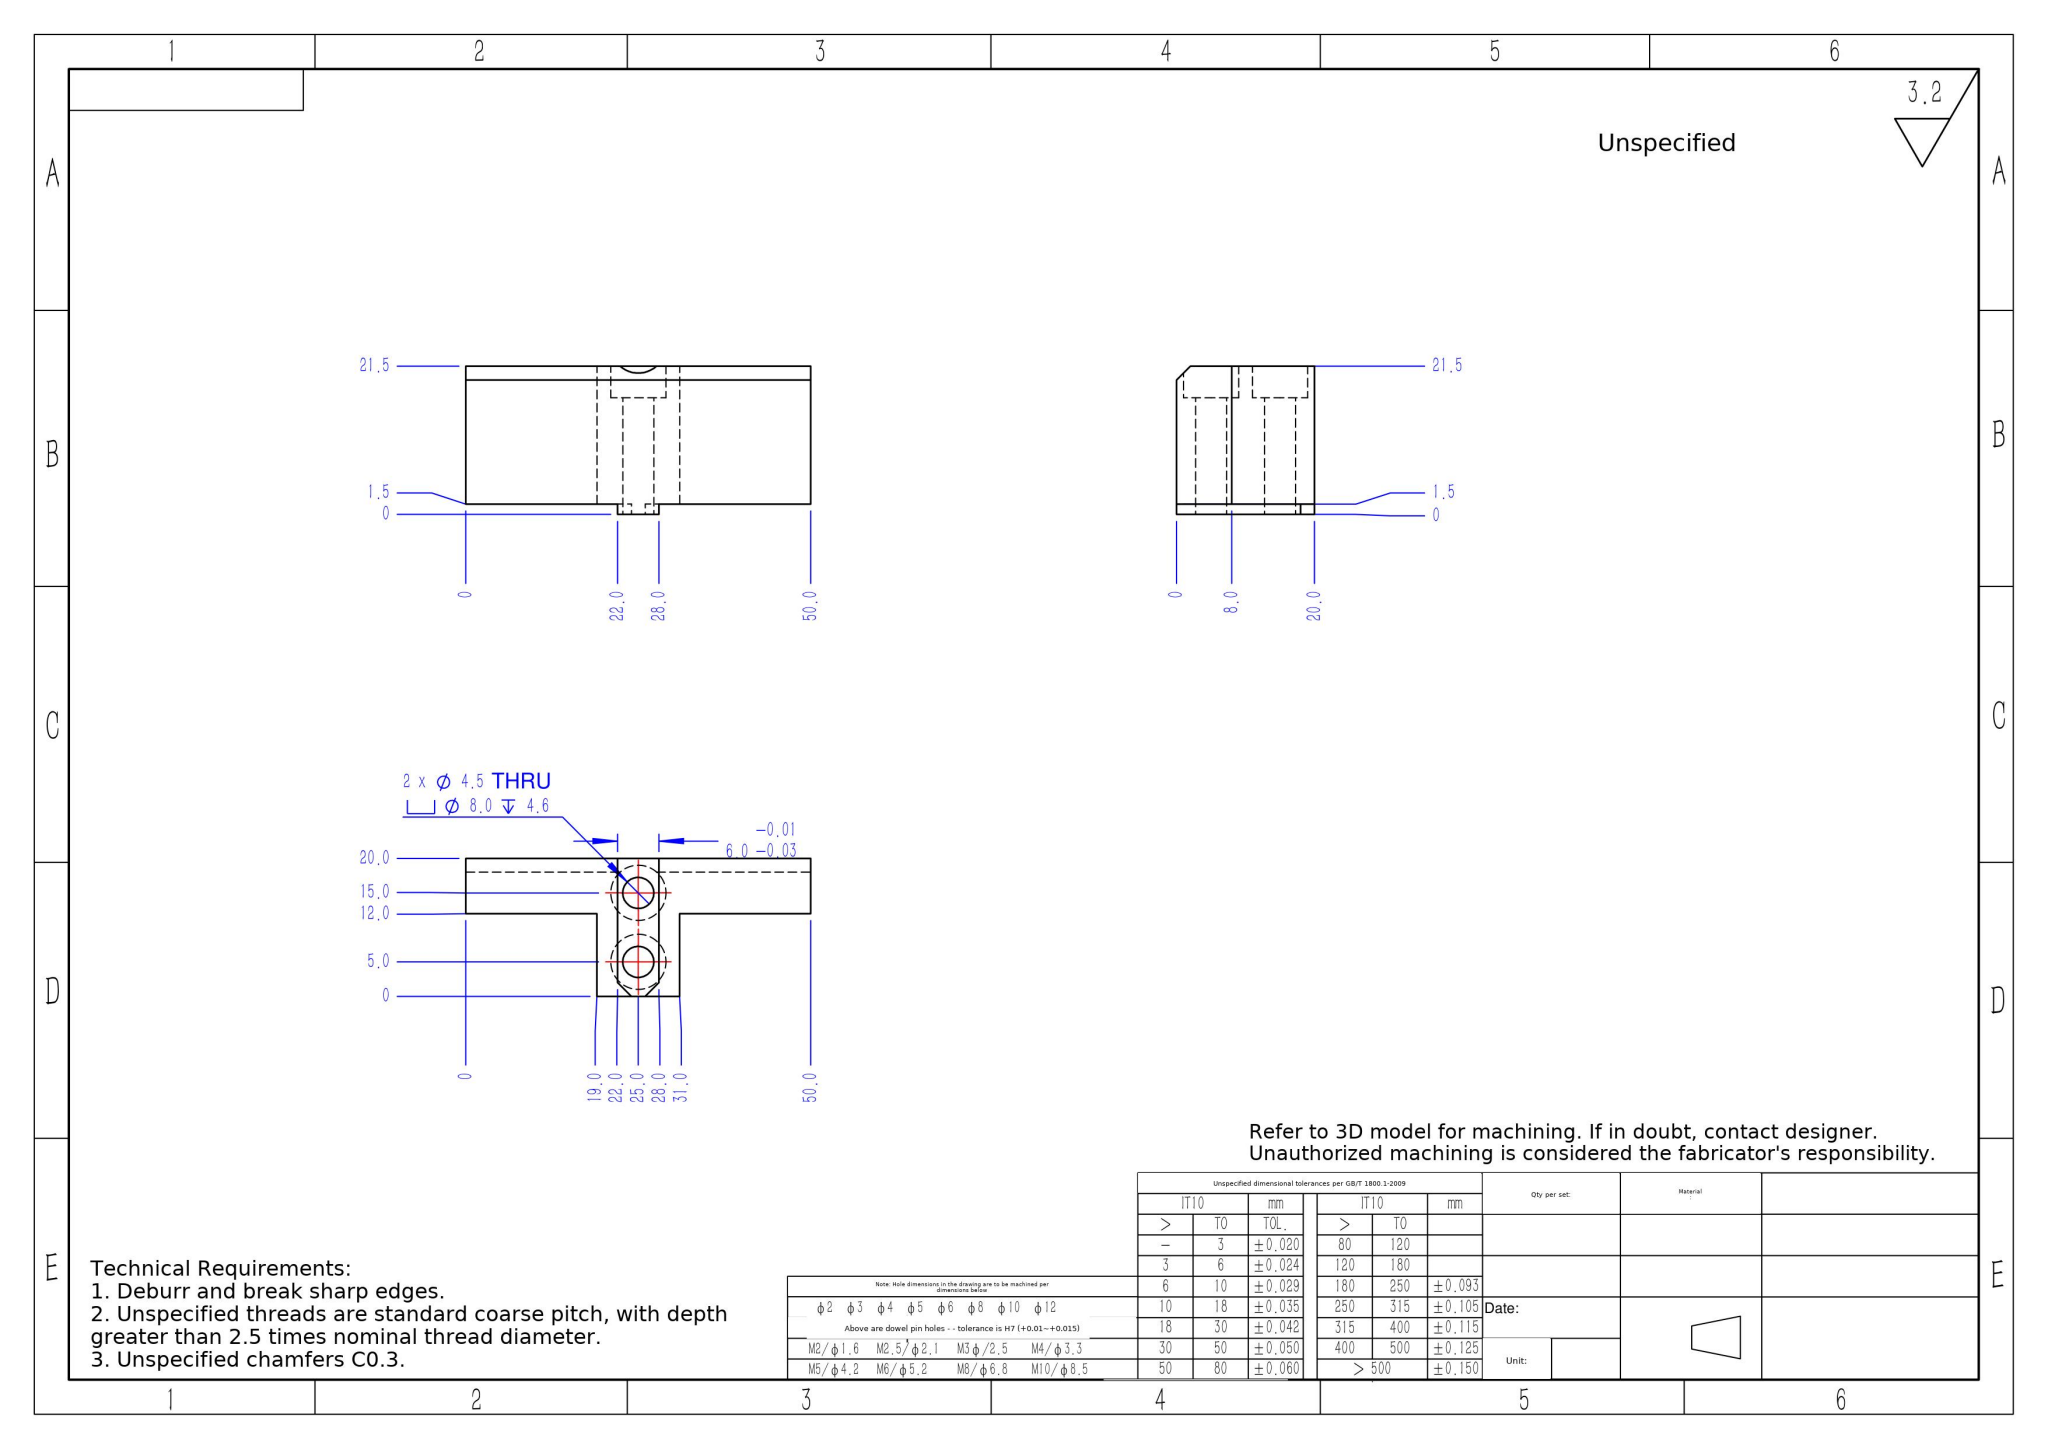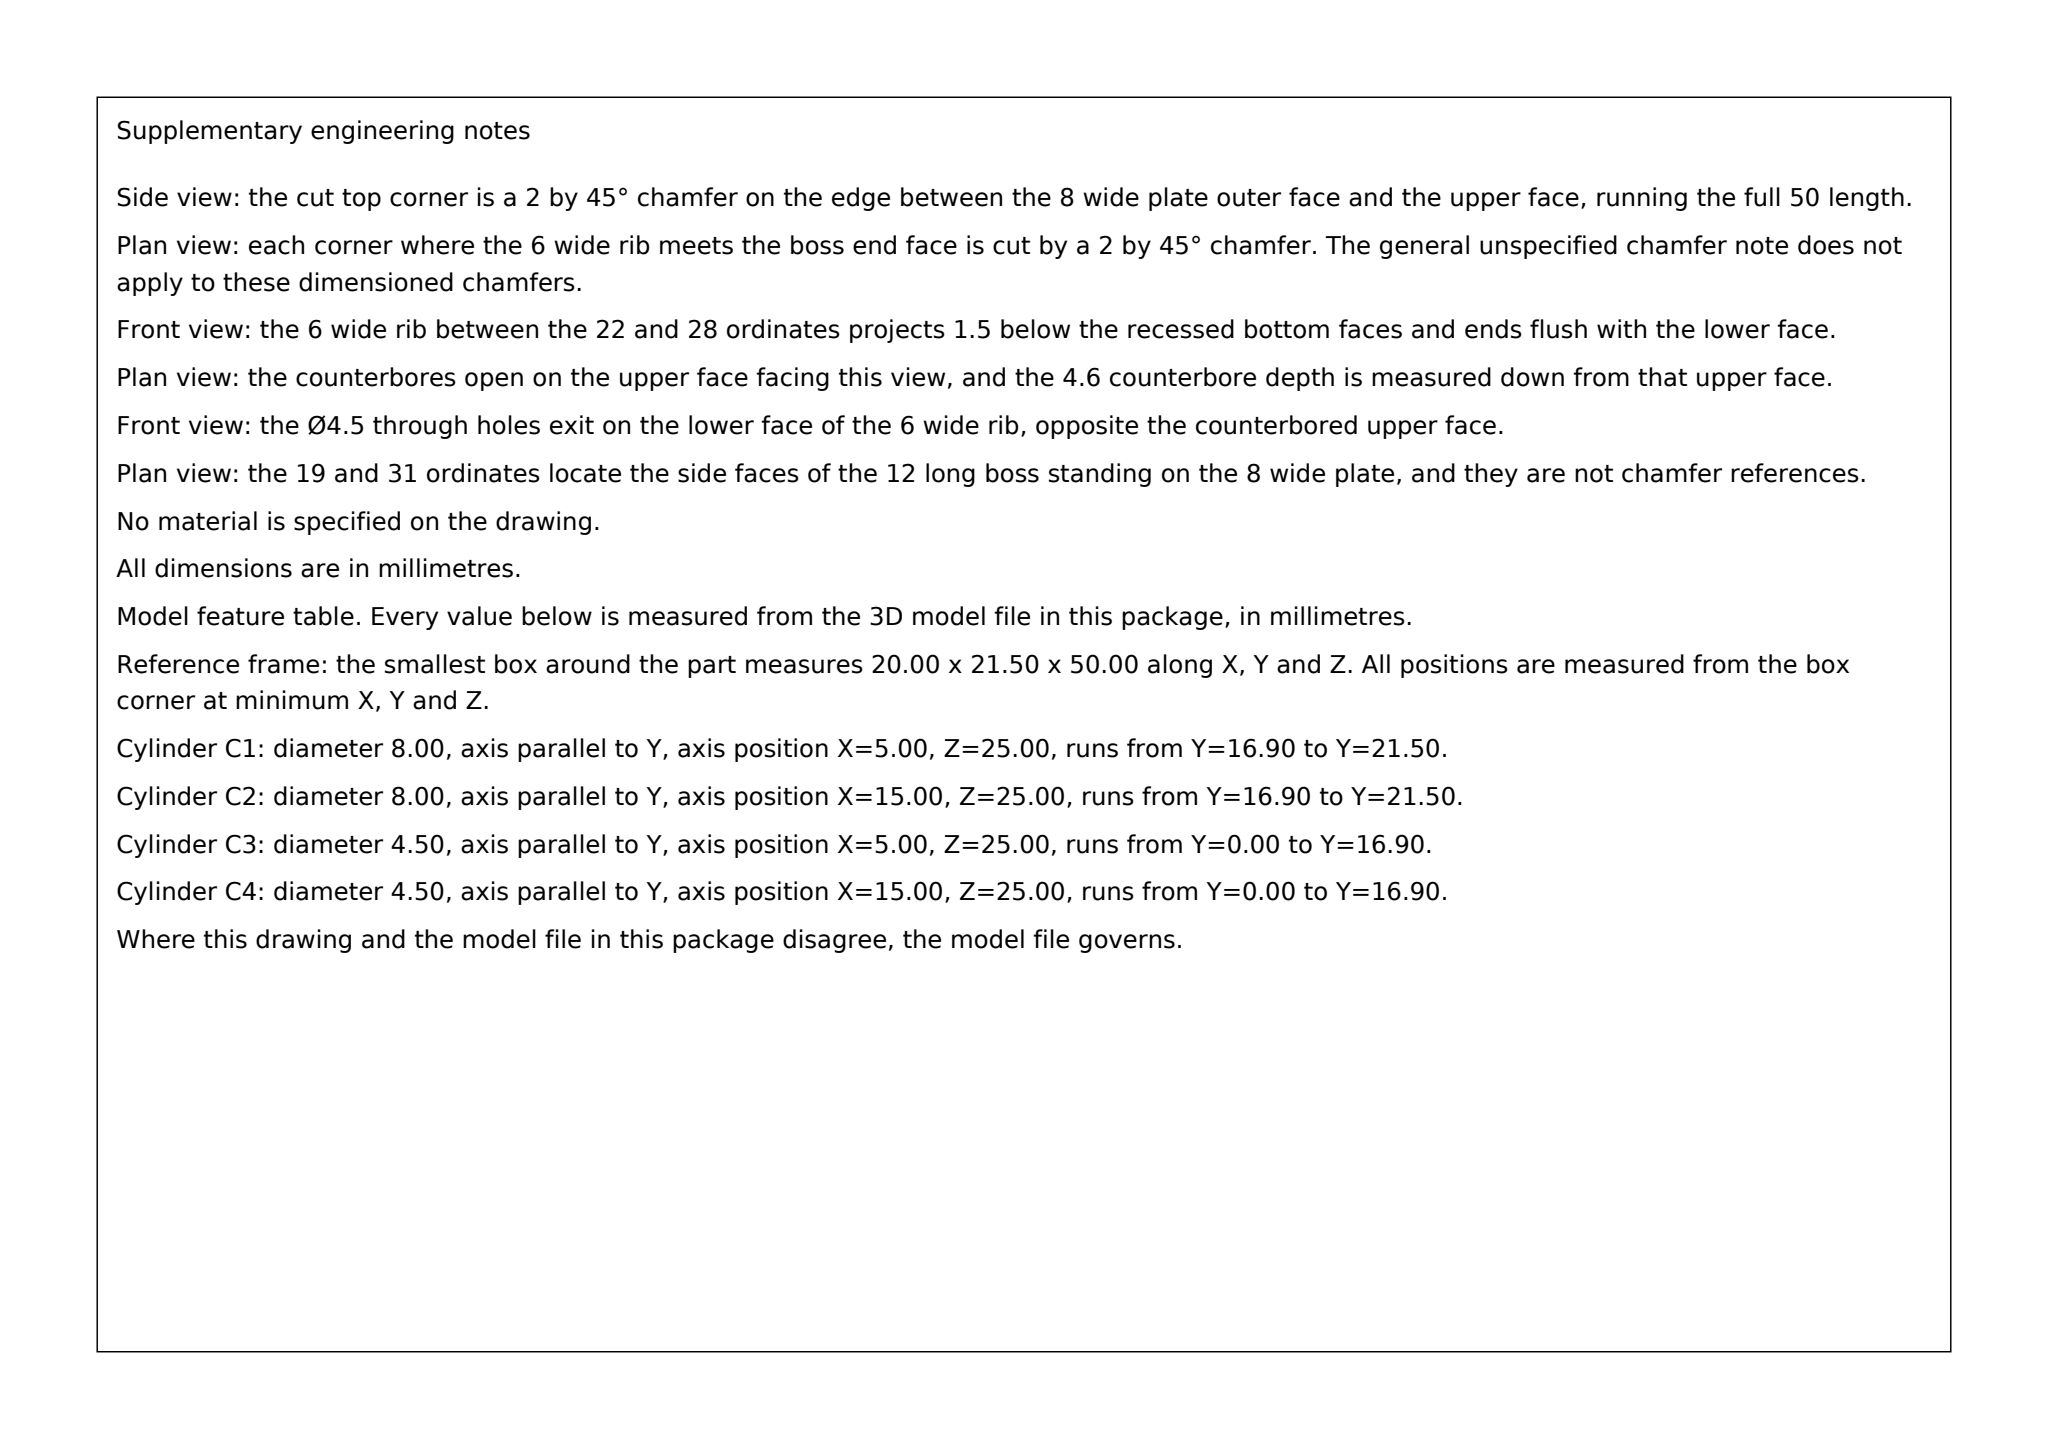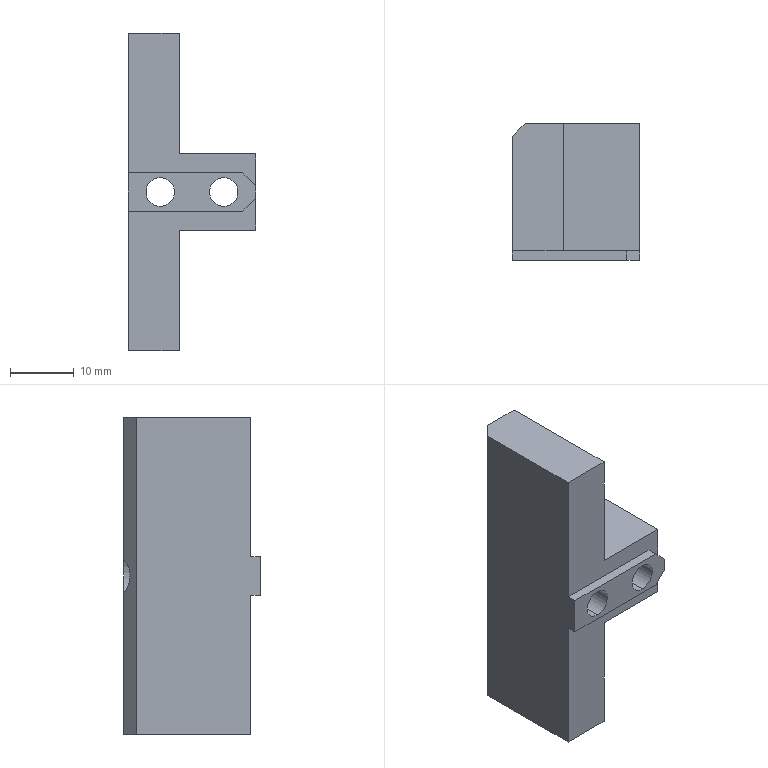Part | SolidWorks | mm | 1 solid | 27 faces | box 20 x 21.5 x 50 mm | volume 9955 mm3 | plane 19 | cylinder 8 | commonest cylinder face diameters 8 x4 4.5 x4
Drawing notes:
2X C2 ON 6 WIDE SLOT ENDS AT 18.0, Z 22.0 & 28.0 | from the solid: inclined_planes 45/90/45 at bbox_from [18,0,22] & [18,0,26], size 2x1.5x2 (two chamfers, 2mm leg = C2) on slot bounded by z=22.0/28.0 faces and x=18 end
STEP:
#1=CARTESIAN_POINT('',(15.,16.9,-29.));
#2=VERTEX_POINT('',#1);
#3=CARTESIAN_POINT('',(15.,16.9,-21.));
#4=VERTEX_POINT('',#3);
#5=CARTESIAN_POINT('',(15.,16.9,-25.));
#6=DIRECTION('',(0.,1.,0.));
#7=DIRECTION('',(0.,0.,1.));
#8=AXIS2_PLACEMENT_3D('',#5,#6,#7);
#9=CIRCLE('',#8,4.);
#10=EDGE_CURVE('',#2,#4,#9,.T.);
#11=ORIENTED_EDGE('',*,*,#10,.F.);
#12=CARTESIAN_POINT('',(15.,21.5,-29.));
#13=VERTEX_POINT('',#12);
#14=CARTESIAN_POINT('',(15.,21.5,-29.));
#15=DIRECTION('',(0.,1.,0.));
#16=VECTOR('',#15,1000.);
#17=LINE('',#14,#16);
#18=EDGE_CURVE('',#2,#13,#17,.T.);
#19=ORIENTED_EDGE('',*,*,#18,.T.);
#20=CARTESIAN_POINT('',(15.,21.5,-21.));
#21=VERTEX_POINT('',#20);
#22=CARTESIAN_POINT('',(15.,21.5,-25.));
#23=DIRECTION('',(0.,1.,0.));
#24=DIRECTION('',(0.,0.,1.));
#25=AXIS2_PLACEMENT_3D('',#22,#23,#24);
#26=CIRCLE('',#25,4.);
#27=EDGE_CURVE('',#13,#21,#26,.T.);
#28=ORIENTED_EDGE('',*,*,#27,.T.);
#29=CARTESIAN_POINT('',(15.,21.5,-21.));
#30=DIRECTION('',(0.,1.,0.));
#31=VECTOR('',#30,1000.);
#32=LINE('',#29,#31);
#33=EDGE_CURVE('',#4,#21,#32,.T.);
#34=ORIENTED_EDGE('',*,*,#33,.F.);
#35=EDGE_LOOP('',(#11,#19,#28,#34));
#36=FACE_OUTER_BOUND('',#35,.T.);
#37=CARTESIAN_POINT('',(15.,21.5,-25.));
#38=DIRECTION('',(0.,1.,0.));
#39=DIRECTION('',(0.,0.,1.));
#40=AXIS2_PLACEMENT_3D('',#37,#38,#39);
#41=CYLINDRICAL_SURFACE('',#40,4.);
#42=ADVANCED_FACE('',(#36),#41,.F.);
#43=CARTESIAN_POINT('',(15.,0.,-27.25));
#44=VERTEX_POINT('',#43);
#45=CARTESIAN_POINT('',(15.,0.,-22.75));
#46=VERTEX_POINT('',#45);
#47=CARTESIAN_POINT('',(15.,0.,-25.));
#48=DIRECTION('',(0.,1.,0.));
#49=DIRECTION('',(0.,0.,1.));
#50=AXIS2_PLACEMENT_3D('',#47,#48,#49);
#51=CIRCLE('',#50,2.25);
#52=EDGE_CURVE('',#44,#46,#51,.T.);
#53=ORIENTED_EDGE('',*,*,#52,.F.);
#54=CARTESIAN_POINT('',(15.,16.9,-27.25));
#55=VERTEX_POINT('',#54);
#56=CARTESIAN_POINT('',(15.,21.5,-27.25));
#57=DIRECTION('',(0.,1.,0.));
#58=VECTOR('',#57,1000.);
#59=LINE('',#56,#58);
#60=EDGE_CURVE('',#44,#55,#59,.T.);
#61=ORIENTED_EDGE('',*,*,#60,.T.);
#62=CARTESIAN_POINT('',(15.,16.9,-22.75));
#63=VERTEX_POINT('',#62);
#64=CARTESIAN_POINT('',(15.,16.9,-25.));
#65=DIRECTION('',(0.,1.,0.));
#66=DIRECTION('',(0.,0.,1.));
#67=AXIS2_PLACEMENT_3D('',#64,#65,#66);
#68=CIRCLE('',#67,2.25);
#69=EDGE_CURVE('',#55,#63,#68,.T.);
#70=ORIENTED_EDGE('',*,*,#69,.T.);
#71=CARTESIAN_POINT('',(15.,21.5,-22.75));
#72=DIRECTION('',(0.,1.,0.));
#73=VECTOR('',#72,1000.);
#74=LINE('',#71,#73);
#75=EDGE_CURVE('',#46,#63,#74,.T.);
#76=ORIENTED_EDGE('',*,*,#75,.F.);
#77=EDGE_LOOP('',(#53,#61,#70,#76));
#78=FACE_OUTER_BOUND('',#77,.T.);
#79=CARTESIAN_POINT('',(15.,21.5,-25.));
#80=DIRECTION('',(0.,1.,0.));
#81=DIRECTION('',(0.,0.,1.));
#82=AXIS2_PLACEMENT_3D('',#79,#80,#81);
#83=CYLINDRICAL_SURFACE('',#82,2.25);
#84=ADVANCED_FACE('',(#78),#83,.F.);
#85=CARTESIAN_POINT('',(5.,16.9,-29.));
#86=VERTEX_POINT('',#85);
#87=CARTESIAN_POINT('',(5.,16.9,-21.));
#88=VERTEX_POINT('',#87);
#89=CARTESIAN_POINT('',(5.,16.9,-25.));
#90=DIRECTION('',(0.,1.,0.));
#91=DIRECTION('',(0.,0.,1.));
#92=AXIS2_PLACEMENT_3D('',#89,#90,#91);
#93=CIRCLE('',#92,4.);
#94=EDGE_CURVE('',#86,#88,#93,.T.);
#95=ORIENTED_EDGE('',*,*,#94,.F.);
#96=CARTESIAN_POINT('',(5.,21.5,-29.));
#97=VERTEX_POINT('',#96);
#98=CARTESIAN_POINT('',(5.,21.5,-29.));
#99=DIRECTION('',(0.,1.,0.));
#100=VECTOR('',#99,1000.);
#101=LINE('',#98,#100);
#102=EDGE_CURVE('',#86,#97,#101,.T.);
#103=ORIENTED_EDGE('',*,*,#102,.T.);
#104=CARTESIAN_POINT('',(2.,21.5,-27.646));
#105=VERTEX_POINT('',#104);
#106=CARTESIAN_POINT('',(5.,21.5,-25.));
#107=DIRECTION('',(0.,1.,0.));
#108=DIRECTION('',(0.,0.,1.));
#109=AXIS2_PLACEMENT_3D('',#106,#107,#108);
#110=CIRCLE('',#109,4.);
#111=EDGE_CURVE('',#97,#105,#110,.T.);
#112=ORIENTED_EDGE('',*,*,#111,.T.);
#113=CARTESIAN_POINT('',(2.,21.5,-22.354));
#114=VERTEX_POINT('',#113);
#115=CARTESIAN_POINT('',(2.,21.5,-27.646));
#116=CARTESIAN_POINT('',(0.6,20.1,-26.058));
#117=CARTESIAN_POINT('',(0.6,20.1,-23.942));
#118=CARTESIAN_POINT('',(2.,21.5,-22.354));
#119=(BOUNDED_CURVE()B_SPLINE_CURVE(3,(#115,#116,#117,#118),.UNSPECIFIED.,.F.,.F.)B_SPLINE_CURVE_WITH_KNOTS((4,4),(2.419,3.864),.UNSPECIFIED.)CURVE()GEOMETRIC_REPRESENTATION_ITEM()RATIONAL_B_SPLINE_CURVE((1.,0.8333,0.8333,1.))REPRESENTATION_ITEM(''));
#120=EDGE_CURVE('',#105,#114,#119,.T.);
#121=ORIENTED_EDGE('',*,*,#120,.T.);
#122=CARTESIAN_POINT('',(5.,21.5,-21.));
#123=VERTEX_POINT('',#122);
#124=CARTESIAN_POINT('',(5.,21.5,-25.));
#125=DIRECTION('',(0.,1.,0.));
#126=DIRECTION('',(0.,0.,1.));
#127=AXIS2_PLACEMENT_3D('',#124,#125,#126);
#128=CIRCLE('',#127,4.);
#129=EDGE_CURVE('',#114,#123,#128,.T.);
#130=ORIENTED_EDGE('',*,*,#129,.T.);
#131=CARTESIAN_POINT('',(5.,21.5,-21.));
#132=DIRECTION('',(0.,1.,0.));
#133=VECTOR('',#132,1000.);
#134=LINE('',#131,#133);
#135=EDGE_CURVE('',#88,#123,#134,.T.);
#136=ORIENTED_EDGE('',*,*,#135,.F.);
#137=EDGE_LOOP('',(#95,#103,#112,#121,#130,#136));
#138=FACE_OUTER_BOUND('',#137,.T.);
#139=CARTESIAN_POINT('',(5.,21.5,-25.));
#140=DIRECTION('',(0.,1.,0.));
#141=DIRECTION('',(0.,0.,1.));
#142=AXIS2_PLACEMENT_3D('',#139,#140,#141);
#143=CYLINDRICAL_SURFACE('',#142,4.);
#144=ADVANCED_FACE('',(#138),#143,.F.);
#145=CARTESIAN_POINT('',(5.,0.,-27.25));
#146=VERTEX_POINT('',#145);
#147=CARTESIAN_POINT('',(5.,0.,-22.75));
#148=VERTEX_POINT('',#147);
#149=CARTESIAN_POINT('',(5.,0.,-25.));
#150=DIRECTION('',(0.,1.,0.));
#151=DIRECTION('',(0.,0.,1.));
#152=AXIS2_PLACEMENT_3D('',#149,#150,#151);
#153=CIRCLE('',#152,2.25);
#154=EDGE_CURVE('',#146,#148,#153,.T.);
#155=ORIENTED_EDGE('',*,*,#154,.F.);
#156=CARTESIAN_POINT('',(5.,16.9,-27.25));
#157=VERTEX_POINT('',#156);
#158=CARTESIAN_POINT('',(5.,21.5,-27.25));
#159=DIRECTION('',(0.,1.,0.));
#160=VECTOR('',#159,1000.);
#161=LINE('',#158,#160);
#162=EDGE_CURVE('',#146,#157,#161,.T.);
#163=ORIENTED_EDGE('',*,*,#162,.T.);
#164=CARTESIAN_POINT('',(5.,16.9,-22.75));
#165=VERTEX_POINT('',#164);
#166=CARTESIAN_POINT('',(5.,16.9,-25.));
#167=DIRECTION('',(0.,1.,0.));
#168=DIRECTION('',(0.,0.,1.));
#169=AXIS2_PLACEMENT_3D('',#166,#167,#168);
#170=CIRCLE('',#169,2.25);
#171=EDGE_CURVE('',#157,#165,#170,.T.);
#172=ORIENTED_EDGE('',*,*,#171,.T.);
#173=CARTESIAN_POINT('',(5.,21.5,-22.75));
#174=DIRECTION('',(0.,1.,0.));
#175=VECTOR('',#174,1000.);
#176=LINE('',#173,#175);
#177=EDGE_CURVE('',#148,#165,#176,.T.);
#178=ORIENTED_EDGE('',*,*,#177,.F.);
#179=EDGE_LOOP('',(#155,#163,#172,#178));
#180=FACE_OUTER_BOUND('',#179,.T.);
#181=CARTESIAN_POINT('',(5.,21.5,-25.));
#182=DIRECTION('',(0.,1.,0.));
#183=DIRECTION('',(0.,0.,1.));
#184=AXIS2_PLACEMENT_3D('',#181,#182,#183);
#185=CYLINDRICAL_SURFACE('',#184,2.25);
#186=ADVANCED_FACE('',(#180),#185,.F.);
#187=CARTESIAN_POINT('',(0.,19.5,0.));
#188=VERTEX_POINT('',#187);
#189=CARTESIAN_POINT('',(0.,1.5,0.));
#190=VERTEX_POINT('',#189);
#191=CARTESIAN_POINT('',(0.,21.5,0.));
#192=DIRECTION('',(0.,-1.,0.));
#193=VECTOR('',#192,1000.);
#194=LINE('',#191,#193);
#195=EDGE_CURVE('',#188,#190,#194,.T.);
#196=ORIENTED_EDGE('',*,*,#195,.F.);
#197=CARTESIAN_POINT('',(0.,19.5,-50.));
#198=VERTEX_POINT('',#197);
#199=CARTESIAN_POINT('',(0.,19.5,0.));
#200=DIRECTION('',(0.,0.,-1.));
#201=VECTOR('',#200,1000.);
#202=LINE('',#199,#201);
#203=EDGE_CURVE('',#188,#198,#202,.T.);
#204=ORIENTED_EDGE('',*,*,#203,.T.);
#205=CARTESIAN_POINT('',(0.,1.5,-50.));
#206=VERTEX_POINT('',#205);
#207=CARTESIAN_POINT('',(0.,21.5,-50.));
#208=DIRECTION('',(0.,-1.,0.));
#209=VECTOR('',#208,1000.);
#210=LINE('',#207,#209);
#211=EDGE_CURVE('',#198,#206,#210,.T.);
#212=ORIENTED_EDGE('',*,*,#211,.T.);
#213=CARTESIAN_POINT('',(0.,1.5,-28.));
#214=VERTEX_POINT('',#213);
#215=CARTESIAN_POINT('',(0.,1.5,-28.));
#216=DIRECTION('',(0.,0.,1.));
#217=VECTOR('',#216,1000.);
#218=LINE('',#215,#217);
#219=EDGE_CURVE('',#206,#214,#218,.T.);
#220=ORIENTED_EDGE('',*,*,#219,.T.);
#221=CARTESIAN_POINT('',(0.,0.,-28.));
#222=VERTEX_POINT('',#221);
#223=CARTESIAN_POINT('',(0.,1.5,-28.));
#224=DIRECTION('',(0.,-1.,0.));
#225=VECTOR('',#224,1000.);
#226=LINE('',#223,#225);
#227=EDGE_CURVE('',#214,#222,#226,.T.);
#228=ORIENTED_EDGE('',*,*,#227,.T.);
#229=CARTESIAN_POINT('',(0.,0.,-22.));
#230=VERTEX_POINT('',#229);
#231=CARTESIAN_POINT('',(0.,0.,0.));
#232=DIRECTION('',(0.,0.,1.));
#233=VECTOR('',#232,1000.);
#234=LINE('',#231,#233);
#235=EDGE_CURVE('',#222,#230,#234,.T.);
#236=ORIENTED_EDGE('',*,*,#235,.T.);
#237=CARTESIAN_POINT('',(0.,1.5,-22.));
#238=VERTEX_POINT('',#237);
#239=CARTESIAN_POINT('',(0.,1.5,-22.));
#240=DIRECTION('',(0.,1.,0.));
#241=VECTOR('',#240,1000.);
#242=LINE('',#239,#241);
#243=EDGE_CURVE('',#230,#238,#242,.T.);
#244=ORIENTED_EDGE('',*,*,#243,.T.);
#245=CARTESIAN_POINT('',(0.,1.5,2.879));
#246=DIRECTION('',(0.,0.,1.));
#247=VECTOR('',#246,1000.);
#248=LINE('',#245,#247);
#249=EDGE_CURVE('',#238,#190,#248,.T.);
#250=ORIENTED_EDGE('',*,*,#249,.T.);
#251=EDGE_LOOP('',(#196,#204,#212,#220,#228,#236,#244,#250));
#252=FACE_OUTER_BOUND('',#251,.T.);
#253=CARTESIAN_POINT('',(0.,21.5,0.));
#254=DIRECTION('',(1.,0.,0.));
#255=DIRECTION('',(0.,0.,-1.));
#256=AXIS2_PLACEMENT_3D('',#253,#254,#255);
#257=PLANE('',#256);
#258=ADVANCED_FACE('',(#252),#257,.F.);
#259=CARTESIAN_POINT('',(2.,21.5,0.));
#260=VERTEX_POINT('',#259);
#261=CARTESIAN_POINT('',(8.,21.5,0.));
#262=VERTEX_POINT('',#261);
#263=CARTESIAN_POINT('',(0.,21.5,0.));
#264=DIRECTION('',(1.,0.,0.));
#265=VECTOR('',#264,1000.);
#266=LINE('',#263,#265);
#267=EDGE_CURVE('',#260,#262,#266,.T.);
#268=ORIENTED_EDGE('',*,*,#267,.F.);
#269=CARTESIAN_POINT('',(2.,21.5,0.));
#270=DIRECTION('',(-0.7071,-0.7071,0.));
#271=VECTOR('',#270,1000.);
#272=LINE('',#269,#271);
#273=EDGE_CURVE('',#260,#188,#272,.T.);
#274=ORIENTED_EDGE('',*,*,#273,.T.);
#275=ORIENTED_EDGE('',*,*,#195,.T.);
#276=CARTESIAN_POINT('',(8.,1.5,0.));
#277=VERTEX_POINT('',#276);
#278=CARTESIAN_POINT('',(0.,1.5,0.));
#279=DIRECTION('',(1.,0.,0.));
#280=VECTOR('',#279,1000.);
#281=LINE('',#278,#280);
#282=EDGE_CURVE('',#190,#277,#281,.T.);
#283=ORIENTED_EDGE('',*,*,#282,.T.);
#284=CARTESIAN_POINT('',(8.,21.5,0.));
#285=DIRECTION('',(0.,1.,0.));
#286=VECTOR('',#285,1000.);
#287=LINE('',#284,#286);
#288=EDGE_CURVE('',#277,#262,#287,.T.);
#289=ORIENTED_EDGE('',*,*,#288,.T.);
#290=EDGE_LOOP('',(#268,#274,#275,#283,#289));
#291=FACE_OUTER_BOUND('',#290,.T.);
#292=CARTESIAN_POINT('',(0.,21.5,0.));
#293=DIRECTION('',(0.,0.,-1.));
#294=DIRECTION('',(-1.,0.,0.));
#295=AXIS2_PLACEMENT_3D('',#292,#293,#294);
#296=PLANE('',#295);
#297=ADVANCED_FACE('',(#291),#296,.F.);
#298=CARTESIAN_POINT('',(20.,1.5,-24.));
#299=VERTEX_POINT('',#298);
#300=CARTESIAN_POINT('',(20.,1.5,-19.));
#301=VERTEX_POINT('',#300);
#302=CARTESIAN_POINT('',(20.,1.5,2.879));
#303=DIRECTION('',(0.,0.,1.));
#304=VECTOR('',#303,1000.);
#305=LINE('',#302,#304);
#306=EDGE_CURVE('',#299,#301,#305,.T.);
#307=ORIENTED_EDGE('',*,*,#306,.F.);
#308=CARTESIAN_POINT('',(20.,0.,-24.));
#309=VERTEX_POINT('',#308);
#310=CARTESIAN_POINT('',(20.,21.5,-24.));
#311=DIRECTION('',(0.,-1.,0.));
#312=VECTOR('',#311,1000.);
#313=LINE('',#310,#312);
#314=EDGE_CURVE('',#299,#309,#313,.T.);
#315=ORIENTED_EDGE('',*,*,#314,.T.);
#316=CARTESIAN_POINT('',(20.,0.,-26.));
#317=VERTEX_POINT('',#316);
#318=CARTESIAN_POINT('',(20.,0.,0.));
#319=DIRECTION('',(0.,0.,-1.));
#320=VECTOR('',#319,1000.);
#321=LINE('',#318,#320);
#322=EDGE_CURVE('',#309,#317,#321,.T.);
#323=ORIENTED_EDGE('',*,*,#322,.T.);
#324=CARTESIAN_POINT('',(20.,1.5,-26.));
#325=VERTEX_POINT('',#324);
#326=CARTESIAN_POINT('',(20.,21.5,-26.));
#327=DIRECTION('',(0.,1.,-0.));
#328=VECTOR('',#327,1000.);
#329=LINE('',#326,#328);
#330=EDGE_CURVE('',#317,#325,#329,.T.);
#331=ORIENTED_EDGE('',*,*,#330,.T.);
#332=CARTESIAN_POINT('',(20.,1.5,-31.));
#333=VERTEX_POINT('',#332);
#334=CARTESIAN_POINT('',(20.,1.5,-28.));
#335=DIRECTION('',(0.,0.,1.));
#336=VECTOR('',#335,1000.);
#337=LINE('',#334,#336);
#338=EDGE_CURVE('',#333,#325,#337,.T.);
#339=ORIENTED_EDGE('',*,*,#338,.F.);
#340=CARTESIAN_POINT('',(20.,21.5,-31.));
#341=VERTEX_POINT('',#340);
#342=CARTESIAN_POINT('',(20.,21.5,-31.));
#343=DIRECTION('',(0.,1.,0.));
#344=VECTOR('',#343,1000.);
#345=LINE('',#342,#344);
#346=EDGE_CURVE('',#333,#341,#345,.T.);
#347=ORIENTED_EDGE('',*,*,#346,.T.);
#348=CARTESIAN_POINT('',(20.,21.5,-19.));
#349=VERTEX_POINT('',#348);
#350=CARTESIAN_POINT('',(20.,21.5,0.));
#351=DIRECTION('',(0.,0.,-1.));
#352=VECTOR('',#351,1000.);
#353=LINE('',#350,#352);
#354=EDGE_CURVE('',#349,#341,#353,.T.);
#355=ORIENTED_EDGE('',*,*,#354,.F.);
#356=CARTESIAN_POINT('',(20.,21.5,-19.));
#357=DIRECTION('',(0.,-1.,0.));
#358=VECTOR('',#357,1000.);
#359=LINE('',#356,#358);
#360=EDGE_CURVE('',#349,#301,#359,.T.);
#361=ORIENTED_EDGE('',*,*,#360,.T.);
#362=EDGE_LOOP('',(#307,#315,#323,#331,#339,#347,#355,#361));
#363=FACE_OUTER_BOUND('',#362,.T.);
#364=CARTESIAN_POINT('',(20.,21.5,0.));
#365=DIRECTION('',(-1.,0.,0.));
#366=DIRECTION('',(0.,0.,1.));
#367=AXIS2_PLACEMENT_3D('',#364,#365,#366);
#368=PLANE('',#367);
#369=ADVANCED_FACE('',(#363),#368,.F.);
#370=ORIENTED_EDGE('',*,*,#211,.F.);
#371=CARTESIAN_POINT('',(2.,21.5,-50.));
#372=VERTEX_POINT('',#371);
#373=CARTESIAN_POINT('',(2.,21.5,-50.));
#374=DIRECTION('',(0.7071,0.7071,0.));
#375=VECTOR('',#374,1000.);
#376=LINE('',#373,#375);
#377=EDGE_CURVE('',#198,#372,#376,.T.);
#378=ORIENTED_EDGE('',*,*,#377,.T.);
#379=CARTESIAN_POINT('',(8.,21.5,-50.));
#380=VERTEX_POINT('',#379);
#381=CARTESIAN_POINT('',(0.,21.5,-50.));
#382=DIRECTION('',(-1.,0.,0.));
#383=VECTOR('',#382,1000.);
#384=LINE('',#381,#383);
#385=EDGE_CURVE('',#380,#372,#384,.T.);
#386=ORIENTED_EDGE('',*,*,#385,.F.);
#387=CARTESIAN_POINT('',(8.,1.5,-50.));
#388=VERTEX_POINT('',#387);
#389=CARTESIAN_POINT('',(8.,21.5,-50.));
#390=DIRECTION('',(0.,-1.,0.));
#391=VECTOR('',#390,1000.);
#392=LINE('',#389,#391);
#393=EDGE_CURVE('',#380,#388,#392,.T.);
#394=ORIENTED_EDGE('',*,*,#393,.T.);
#395=CARTESIAN_POINT('',(0.,1.5,-50.));
#396=DIRECTION('',(-1.,0.,0.));
#397=VECTOR('',#396,1000.);
#398=LINE('',#395,#397);
#399=EDGE_CURVE('',#388,#206,#398,.T.);
#400=ORIENTED_EDGE('',*,*,#399,.T.);
#401=EDGE_LOOP('',(#370,#378,#386,#394,#400));
#402=FACE_OUTER_BOUND('',#401,.T.);
#403=CARTESIAN_POINT('',(0.,21.5,-50.));
#404=DIRECTION('',(0.,0.,1.));
#405=DIRECTION('',(1.,0.,0.));
#406=AXIS2_PLACEMENT_3D('',#403,#404,#405);
#407=PLANE('',#406);
#408=ADVANCED_FACE('',(#402),#407,.F.);
#409=CARTESIAN_POINT('',(15.,21.5,-25.));
#410=DIRECTION('',(0.,1.,0.));
#411=DIRECTION('',(0.,0.,1.));
#412=AXIS2_PLACEMENT_3D('',#409,#410,#411);
#413=CIRCLE('',#412,4.);
#414=EDGE_CURVE('',#21,#13,#413,.T.);
#415=ORIENTED_EDGE('',*,*,#414,.F.);
#416=ORIENTED_EDGE('',*,*,#27,.F.);
#417=EDGE_LOOP('',(#415,#416));
#418=FACE_BOUND('',#417,.T.);
#419=ORIENTED_EDGE('',*,*,#385,.T.);
#420=CARTESIAN_POINT('',(2.,21.5,0.));
#421=DIRECTION('',(0.,0.,1.));
#422=VECTOR('',#421,1000.);
#423=LINE('',#420,#422);
#424=EDGE_CURVE('',#372,#105,#423,.T.);
#425=ORIENTED_EDGE('',*,*,#424,.T.);
#426=ORIENTED_EDGE('',*,*,#111,.F.);
#427=CARTESIAN_POINT('',(5.,21.5,-25.));
#428=DIRECTION('',(0.,1.,0.));
#429=DIRECTION('',(0.,0.,1.));
#430=AXIS2_PLACEMENT_3D('',#427,#428,#429);
#431=CIRCLE('',#430,4.);
#432=EDGE_CURVE('',#123,#97,#431,.T.);
#433=ORIENTED_EDGE('',*,*,#432,.F.);
#434=ORIENTED_EDGE('',*,*,#129,.F.);
#435=CARTESIAN_POINT('',(2.,21.5,0.));
#436=DIRECTION('',(0.,0.,1.));
#437=VECTOR('',#436,1000.);
#438=LINE('',#435,#437);
#439=EDGE_CURVE('',#114,#260,#438,.T.);
#440=ORIENTED_EDGE('',*,*,#439,.T.);
#441=ORIENTED_EDGE('',*,*,#267,.T.);
#442=CARTESIAN_POINT('',(8.,21.5,-19.));
#443=VERTEX_POINT('',#442);
#444=CARTESIAN_POINT('',(8.,21.5,10.159));
#445=DIRECTION('',(0.,0.,1.));
#446=VECTOR('',#445,1000.);
#447=LINE('',#444,#446);
#448=EDGE_CURVE('',#443,#262,#447,.T.);
#449=ORIENTED_EDGE('',*,*,#448,.F.);
#450=CARTESIAN_POINT('',(8.,21.5,-19.));
#451=DIRECTION('',(-1.,0.,0.));
#452=VECTOR('',#451,1000.);
#453=LINE('',#450,#452);
#454=EDGE_CURVE('',#349,#443,#453,.T.);
#455=ORIENTED_EDGE('',*,*,#454,.F.);
#456=ORIENTED_EDGE('',*,*,#354,.T.);
#457=CARTESIAN_POINT('',(8.,21.5,-31.));
#458=VERTEX_POINT('',#457);
#459=CARTESIAN_POINT('',(8.,21.5,-31.));
#460=DIRECTION('',(1.,0.,0.));
#461=VECTOR('',#460,1000.);
#462=LINE('',#459,#461);
#463=EDGE_CURVE('',#458,#341,#462,.T.);
#464=ORIENTED_EDGE('',*,*,#463,.F.);
#465=CARTESIAN_POINT('',(8.,21.5,-50.245));
#466=DIRECTION('',(0.,0.,1.));
#467=VECTOR('',#466,1000.);
#468=LINE('',#465,#467);
#469=EDGE_CURVE('',#380,#458,#468,.T.);
#470=ORIENTED_EDGE('',*,*,#469,.F.);
#471=EDGE_LOOP('',(#419,#425,#426,#433,#434,#440,#441,#449,#455,#456,#464,#470));
#472=FACE_OUTER_BOUND('',#471,.T.);
#473=CARTESIAN_POINT('',(0.,21.5,0.));
#474=DIRECTION('',(0.,-1.,0.));
#475=DIRECTION('',(0.,0.,-1.));
#476=AXIS2_PLACEMENT_3D('',#473,#474,#475);
#477=PLANE('',#476);
#478=ADVANCED_FACE('',(#418,#472),#477,.F.);
#479=CARTESIAN_POINT('',(15.,0.,-25.));
#480=DIRECTION('',(0.,1.,0.));
#481=DIRECTION('',(0.,0.,1.));
#482=AXIS2_PLACEMENT_3D('',#479,#480,#481);
#483=CIRCLE('',#482,2.25);
#484=EDGE_CURVE('',#46,#44,#483,.T.);
#485=ORIENTED_EDGE('',*,*,#484,.T.);
#486=ORIENTED_EDGE('',*,*,#52,.T.);
#487=EDGE_LOOP('',(#485,#486));
#488=FACE_BOUND('',#487,.T.);
#489=CARTESIAN_POINT('',(5.,0.,-25.));
#490=DIRECTION('',(0.,1.,0.));
#491=DIRECTION('',(0.,0.,1.));
#492=AXIS2_PLACEMENT_3D('',#489,#490,#491);
#493=CIRCLE('',#492,2.25);
#494=EDGE_CURVE('',#148,#146,#493,.T.);
#495=ORIENTED_EDGE('',*,*,#494,.T.);
#496=ORIENTED_EDGE('',*,*,#154,.T.);
#497=EDGE_LOOP('',(#495,#496));
#498=FACE_BOUND('',#497,.T.);
#499=ORIENTED_EDGE('',*,*,#322,.F.);
#500=CARTESIAN_POINT('',(18.,0.,-22.));
#501=VERTEX_POINT('',#500);
#502=CARTESIAN_POINT('',(-2.,0.,-2.));
#503=DIRECTION('',(-0.7071,0.,0.7071));
#504=VECTOR('',#503,1000.);
#505=LINE('',#502,#504);
#506=EDGE_CURVE('',#309,#501,#505,.T.);
#507=ORIENTED_EDGE('',*,*,#506,.T.);
#508=CARTESIAN_POINT('',(0.,0.,-22.));
#509=DIRECTION('',(1.,0.,0.));
#510=VECTOR('',#509,1000.);
#511=LINE('',#508,#510);
#512=EDGE_CURVE('',#230,#501,#511,.T.);
#513=ORIENTED_EDGE('',*,*,#512,.F.);
#514=ORIENTED_EDGE('',*,*,#235,.F.);
#515=CARTESIAN_POINT('',(18.,0.,-28.));
#516=VERTEX_POINT('',#515);
#517=CARTESIAN_POINT('',(0.,0.,-28.));
#518=DIRECTION('',(-1.,0.,0.));
#519=VECTOR('',#518,1000.);
#520=LINE('',#517,#519);
#521=EDGE_CURVE('',#516,#222,#520,.T.);
#522=ORIENTED_EDGE('',*,*,#521,.F.);
#523=CARTESIAN_POINT('',(23.,0.,-23.));
#524=DIRECTION('',(0.7071,0.,0.7071));
#525=VECTOR('',#524,1000.);
#526=LINE('',#523,#525);
#527=EDGE_CURVE('',#516,#317,#526,.T.);
#528=ORIENTED_EDGE('',*,*,#527,.T.);
#529=EDGE_LOOP('',(#499,#507,#513,#514,#522,#528));
#530=FACE_OUTER_BOUND('',#529,.T.);
#531=CARTESIAN_POINT('',(0.,0.,0.));
#532=DIRECTION('',(0.,-1.,0.));
#533=DIRECTION('',(0.,0.,-1.));
#534=AXIS2_PLACEMENT_3D('',#531,#532,#533);
#535=PLANE('',#534);
#536=ADVANCED_FACE('',(#488,#498,#530),#535,.T.);
#537=CARTESIAN_POINT('',(8.,1.5,-19.));
#538=VERTEX_POINT('',#537);
#539=CARTESIAN_POINT('',(0.,1.5,-19.));
#540=DIRECTION('',(-1.,0.,0.));
#541=VECTOR('',#540,1000.);
#542=LINE('',#539,#541);
#543=EDGE_CURVE('',#301,#538,#542,.T.);
#544=ORIENTED_EDGE('',*,*,#543,.T.);
#545=CARTESIAN_POINT('',(8.,1.5,2.879));
#546=DIRECTION('',(0.,0.,1.));
#547=VECTOR('',#546,1000.);
#548=LINE('',#545,#547);
#549=EDGE_CURVE('',#538,#277,#548,.T.);
#550=ORIENTED_EDGE('',*,*,#549,.T.);
#551=ORIENTED_EDGE('',*,*,#282,.F.);
#552=ORIENTED_EDGE('',*,*,#249,.F.);
#553=CARTESIAN_POINT('',(18.,1.5,-22.));
#554=VERTEX_POINT('',#553);
#555=CARTESIAN_POINT('',(0.,1.5,-22.));
#556=DIRECTION('',(1.,0.,0.));
#557=VECTOR('',#556,1000.);
#558=LINE('',#555,#557);
#559=EDGE_CURVE('',#238,#554,#558,.T.);
#560=ORIENTED_EDGE('',*,*,#559,.T.);
#561=CARTESIAN_POINT('',(-3.44,1.5,-0.5604));
#562=DIRECTION('',(0.7071,0.,-0.7071));
#563=VECTOR('',#562,1000.);
#564=LINE('',#561,#563);
#565=EDGE_CURVE('',#554,#299,#564,.T.);
#566=ORIENTED_EDGE('',*,*,#565,.T.);
#567=ORIENTED_EDGE('',*,*,#306,.T.);
#568=EDGE_LOOP('',(#544,#550,#551,#552,#560,#566,#567));
#569=FACE_OUTER_BOUND('',#568,.T.);
#570=CARTESIAN_POINT('',(0.,1.5,2.879));
#571=DIRECTION('',(0.,1.,0.));
#572=DIRECTION('',(0.,0.,1.));
#573=AXIS2_PLACEMENT_3D('',#570,#571,#572);
#574=PLANE('',#573);
#575=ADVANCED_FACE('',(#569),#574,.F.);
#576=ORIENTED_EDGE('',*,*,#512,.T.);
#577=CARTESIAN_POINT('',(18.,1.5,-22.));
#578=DIRECTION('',(0.,1.,0.));
#579=VECTOR('',#578,1000.);
#580=LINE('',#577,#579);
#581=EDGE_CURVE('',#501,#554,#580,.T.);
#582=ORIENTED_EDGE('',*,*,#581,.T.);
#583=ORIENTED_EDGE('',*,*,#559,.F.);
#584=ORIENTED_EDGE('',*,*,#243,.F.);
#585=EDGE_LOOP('',(#576,#582,#583,#584));
#586=FACE_OUTER_BOUND('',#585,.T.);
#587=CARTESIAN_POINT('',(0.,1.5,-22.));
#588=DIRECTION('',(0.,0.,-1.));
#589=DIRECTION('',(-1.,0.,0.));
#590=AXIS2_PLACEMENT_3D('',#587,#588,#589);
#591=PLANE('',#590);
#592=ADVANCED_FACE('',(#586),#591,.F.);
#593=ORIENTED_EDGE('',*,*,#399,.F.);
#594=CARTESIAN_POINT('',(8.,1.5,-31.));
#595=VERTEX_POINT('',#594);
#596=CARTESIAN_POINT('',(8.,1.5,-28.));
#597=DIRECTION('',(0.,0.,1.));
#598=VECTOR('',#597,1000.);
#599=LINE('',#596,#598);
#600=EDGE_CURVE('',#388,#595,#599,.T.);
#601=ORIENTED_EDGE('',*,*,#600,.T.);
#602=CARTESIAN_POINT('',(0.,1.5,-31.));
#603=DIRECTION('',(1.,0.,0.));
#604=VECTOR('',#603,1000.);
#605=LINE('',#602,#604);
#606=EDGE_CURVE('',#595,#333,#605,.T.);
#607=ORIENTED_EDGE('',*,*,#606,.T.);
#608=ORIENTED_EDGE('',*,*,#338,.T.);
#609=CARTESIAN_POINT('',(18.,1.5,-28.));
#610=VERTEX_POINT('',#609);
#611=CARTESIAN_POINT('',(9.,1.5,-37.));
#612=DIRECTION('',(-0.7071,0.,-0.7071));
#613=VECTOR('',#612,1000.);
#614=LINE('',#611,#613);
#615=EDGE_CURVE('',#325,#610,#614,.T.);
#616=ORIENTED_EDGE('',*,*,#615,.T.);
#617=CARTESIAN_POINT('',(0.,1.5,-28.));
#618=DIRECTION('',(1.,0.,0.));
#619=VECTOR('',#618,1000.);
#620=LINE('',#617,#619);
#621=EDGE_CURVE('',#214,#610,#620,.T.);
#622=ORIENTED_EDGE('',*,*,#621,.F.);
#623=ORIENTED_EDGE('',*,*,#219,.F.);
#624=EDGE_LOOP('',(#593,#601,#607,#608,#616,#622,#623));
#625=FACE_OUTER_BOUND('',#624,.T.);
#626=CARTESIAN_POINT('',(0.,1.5,-28.));
#627=DIRECTION('',(0.,1.,0.));
#628=DIRECTION('',(0.,0.,1.));
#629=AXIS2_PLACEMENT_3D('',#626,#627,#628);
#630=PLANE('',#629);
#631=ADVANCED_FACE('',(#625),#630,.F.);
#632=ORIENTED_EDGE('',*,*,#621,.T.);
#633=CARTESIAN_POINT('',(18.,1.5,-28.));
#634=DIRECTION('',(0.,-1.,0.));
#635=VECTOR('',#634,1000.);
#636=LINE('',#633,#635);
#637=EDGE_CURVE('',#610,#516,#636,.T.);
#638=ORIENTED_EDGE('',*,*,#637,.T.);
#639=ORIENTED_EDGE('',*,*,#521,.T.);
#640=ORIENTED_EDGE('',*,*,#227,.F.);
#641=EDGE_LOOP('',(#632,#638,#639,#640));
#642=FACE_OUTER_BOUND('',#641,.T.);
#643=CARTESIAN_POINT('',(0.,1.5,-28.));
#644=DIRECTION('',(0.,0.,1.));
#645=DIRECTION('',(0.,-1.,0.));
#646=AXIS2_PLACEMENT_3D('',#643,#644,#645);
#647=PLANE('',#646);
#648=ADVANCED_FACE('',(#642),#647,.F.);
#649=ORIENTED_EDGE('',*,*,#469,.T.);
#650=CARTESIAN_POINT('',(8.,0.,-31.));
#651=DIRECTION('',(0.,1.,0.));
#652=VECTOR('',#651,1000.);
#653=LINE('',#650,#652);
#654=EDGE_CURVE('',#595,#458,#653,.T.);
#655=ORIENTED_EDGE('',*,*,#654,.F.);
#656=ORIENTED_EDGE('',*,*,#600,.F.);
#657=ORIENTED_EDGE('',*,*,#393,.F.);
#658=EDGE_LOOP('',(#649,#655,#656,#657));
#659=FACE_OUTER_BOUND('',#658,.T.);
#660=CARTESIAN_POINT('',(8.,0.,-50.245));
#661=DIRECTION('',(-1.,0.,0.));
#662=DIRECTION('',(0.,0.,1.));
#663=AXIS2_PLACEMENT_3D('',#660,#661,#662);
#664=PLANE('',#663);
#665=ADVANCED_FACE('',(#659),#664,.F.);
#666=ORIENTED_EDGE('',*,*,#606,.F.);
#667=ORIENTED_EDGE('',*,*,#654,.T.);
#668=ORIENTED_EDGE('',*,*,#463,.T.);
#669=ORIENTED_EDGE('',*,*,#346,.F.);
#670=EDGE_LOOP('',(#666,#667,#668,#669));
#671=FACE_OUTER_BOUND('',#670,.T.);
#672=CARTESIAN_POINT('',(8.,0.,-31.));
#673=DIRECTION('',(0.,0.,1.));
#674=DIRECTION('',(1.,0.,0.));
#675=AXIS2_PLACEMENT_3D('',#672,#673,#674);
#676=PLANE('',#675);
#677=ADVANCED_FACE('',(#671),#676,.F.);
#678=ORIENTED_EDGE('',*,*,#549,.F.);
#679=CARTESIAN_POINT('',(8.,0.,-19.));
#680=DIRECTION('',(0.,1.,0.));
#681=VECTOR('',#680,1000.);
#682=LINE('',#679,#681);
#683=EDGE_CURVE('',#538,#443,#682,.T.);
#684=ORIENTED_EDGE('',*,*,#683,.T.);
#685=ORIENTED_EDGE('',*,*,#448,.T.);
#686=ORIENTED_EDGE('',*,*,#288,.F.);
#687=EDGE_LOOP('',(#678,#684,#685,#686));
#688=FACE_OUTER_BOUND('',#687,.T.);
#689=CARTESIAN_POINT('',(8.,0.,10.159));
#690=DIRECTION('',(-1.,0.,0.));
#691=DIRECTION('',(0.,0.,1.));
#692=AXIS2_PLACEMENT_3D('',#689,#690,#691);
#693=PLANE('',#692);
#694=ADVANCED_FACE('',(#688),#693,.F.);
#695=ORIENTED_EDGE('',*,*,#454,.T.);
#696=ORIENTED_EDGE('',*,*,#683,.F.);
#697=ORIENTED_EDGE('',*,*,#543,.F.);
#698=ORIENTED_EDGE('',*,*,#360,.F.);
#699=EDGE_LOOP('',(#695,#696,#697,#698));
#700=FACE_OUTER_BOUND('',#699,.T.);
#701=CARTESIAN_POINT('',(8.,0.,-19.));
#702=DIRECTION('',(0.,0.,-1.));
#703=DIRECTION('',(-1.,0.,0.));
#704=AXIS2_PLACEMENT_3D('',#701,#702,#703);
#705=PLANE('',#704);
#706=ADVANCED_FACE('',(#700),#705,.F.);
#707=ORIENTED_EDGE('',*,*,#162,.F.);
#708=ORIENTED_EDGE('',*,*,#494,.F.);
#709=ORIENTED_EDGE('',*,*,#177,.T.);
#710=CARTESIAN_POINT('',(5.,16.9,-25.));
#711=DIRECTION('',(0.,1.,0.));
#712=DIRECTION('',(0.,0.,1.));
#713=AXIS2_PLACEMENT_3D('',#710,#711,#712);
#714=CIRCLE('',#713,2.25);
#715=EDGE_CURVE('',#165,#157,#714,.T.);
#716=ORIENTED_EDGE('',*,*,#715,.T.);
#717=EDGE_LOOP('',(#707,#708,#709,#716));
#718=FACE_OUTER_BOUND('',#717,.T.);
#719=CARTESIAN_POINT('',(5.,21.5,-25.));
#720=DIRECTION('',(0.,1.,0.));
#721=DIRECTION('',(0.,0.,1.));
#722=AXIS2_PLACEMENT_3D('',#719,#720,#721);
#723=CYLINDRICAL_SURFACE('',#722,2.25);
#724=ADVANCED_FACE('',(#718),#723,.F.);
#725=ORIENTED_EDGE('',*,*,#715,.F.);
#726=ORIENTED_EDGE('',*,*,#171,.F.);
#727=EDGE_LOOP('',(#725,#726));
#728=FACE_BOUND('',#727,.T.);
#729=CARTESIAN_POINT('',(5.,16.9,-25.));
#730=DIRECTION('',(0.,1.,0.));
#731=DIRECTION('',(0.,0.,1.));
#732=AXIS2_PLACEMENT_3D('',#729,#730,#731);
#733=CIRCLE('',#732,4.);
#734=EDGE_CURVE('',#88,#86,#733,.T.);
#735=ORIENTED_EDGE('',*,*,#734,.T.);
#736=ORIENTED_EDGE('',*,*,#94,.T.);
#737=EDGE_LOOP('',(#735,#736));
#738=FACE_OUTER_BOUND('',#737,.T.);
#739=CARTESIAN_POINT('',(7.25,16.9,-25.));
#740=DIRECTION('',(0.,-1.,0.));
#741=DIRECTION('',(0.,0.,-1.));
#742=AXIS2_PLACEMENT_3D('',#739,#740,#741);
#743=PLANE('',#742);
#744=ADVANCED_FACE('',(#728,#738),#743,.F.);
#745=ORIENTED_EDGE('',*,*,#102,.F.);
#746=ORIENTED_EDGE('',*,*,#734,.F.);
#747=ORIENTED_EDGE('',*,*,#135,.T.);
#748=ORIENTED_EDGE('',*,*,#432,.T.);
#749=EDGE_LOOP('',(#745,#746,#747,#748));
#750=FACE_OUTER_BOUND('',#749,.T.);
#751=CARTESIAN_POINT('',(5.,21.5,-25.));
#752=DIRECTION('',(0.,1.,0.));
#753=DIRECTION('',(0.,0.,1.));
#754=AXIS2_PLACEMENT_3D('',#751,#752,#753);
#755=CYLINDRICAL_SURFACE('',#754,4.);
#756=ADVANCED_FACE('',(#750),#755,.F.);
#757=ORIENTED_EDGE('',*,*,#60,.F.);
#758=ORIENTED_EDGE('',*,*,#484,.F.);
#759=ORIENTED_EDGE('',*,*,#75,.T.);
#760=CARTESIAN_POINT('',(15.,16.9,-25.));
#761=DIRECTION('',(0.,1.,0.));
#762=DIRECTION('',(0.,0.,1.));
#763=AXIS2_PLACEMENT_3D('',#760,#761,#762);
#764=CIRCLE('',#763,2.25);
#765=EDGE_CURVE('',#63,#55,#764,.T.);
#766=ORIENTED_EDGE('',*,*,#765,.T.);
#767=EDGE_LOOP('',(#757,#758,#759,#766));
#768=FACE_OUTER_BOUND('',#767,.T.);
#769=CARTESIAN_POINT('',(15.,21.5,-25.));
#770=DIRECTION('',(0.,1.,0.));
#771=DIRECTION('',(0.,0.,1.));
#772=AXIS2_PLACEMENT_3D('',#769,#770,#771);
#773=CYLINDRICAL_SURFACE('',#772,2.25);
#774=ADVANCED_FACE('',(#768),#773,.F.);
#775=ORIENTED_EDGE('',*,*,#765,.F.);
#776=ORIENTED_EDGE('',*,*,#69,.F.);
#777=EDGE_LOOP('',(#775,#776));
#778=FACE_BOUND('',#777,.T.);
#779=CARTESIAN_POINT('',(15.,16.9,-25.));
#780=DIRECTION('',(0.,1.,0.));
#781=DIRECTION('',(0.,0.,1.));
#782=AXIS2_PLACEMENT_3D('',#779,#780,#781);
#783=CIRCLE('',#782,4.);
#784=EDGE_CURVE('',#4,#2,#783,.T.);
#785=ORIENTED_EDGE('',*,*,#784,.T.);
#786=ORIENTED_EDGE('',*,*,#10,.T.);
#787=EDGE_LOOP('',(#785,#786));
#788=FACE_OUTER_BOUND('',#787,.T.);
#789=CARTESIAN_POINT('',(17.25,16.9,-25.));
#790=DIRECTION('',(0.,-1.,0.));
#791=DIRECTION('',(0.,0.,-1.));
#792=AXIS2_PLACEMENT_3D('',#789,#790,#791);
#793=PLANE('',#792);
#794=ADVANCED_FACE('',(#778,#788),#793,.F.);
#795=ORIENTED_EDGE('',*,*,#18,.F.);
#796=ORIENTED_EDGE('',*,*,#784,.F.);
#797=ORIENTED_EDGE('',*,*,#33,.T.);
#798=ORIENTED_EDGE('',*,*,#414,.T.);
#799=EDGE_LOOP('',(#795,#796,#797,#798));
#800=FACE_OUTER_BOUND('',#799,.T.);
#801=CARTESIAN_POINT('',(15.,21.5,-25.));
#802=DIRECTION('',(0.,1.,0.));
#803=DIRECTION('',(0.,0.,1.));
#804=AXIS2_PLACEMENT_3D('',#801,#802,#803);
#805=CYLINDRICAL_SURFACE('',#804,4.);
#806=ADVANCED_FACE('',(#800),#805,.F.);
#807=ORIENTED_EDGE('',*,*,#377,.F.);
#808=ORIENTED_EDGE('',*,*,#203,.F.);
#809=ORIENTED_EDGE('',*,*,#273,.F.);
#810=ORIENTED_EDGE('',*,*,#439,.F.);
#811=ORIENTED_EDGE('',*,*,#120,.F.);
#812=ORIENTED_EDGE('',*,*,#424,.F.);
#813=EDGE_LOOP('',(#807,#808,#809,#810,#811,#812));
#814=FACE_OUTER_BOUND('',#813,.T.);
#815=CARTESIAN_POINT('',(2.,21.5,0.));
#816=DIRECTION('',(0.7071,-0.7071,0.));
#817=DIRECTION('',(0.,0.,1.));
#818=AXIS2_PLACEMENT_3D('',#815,#816,#817);
#819=PLANE('',#818);
#820=ADVANCED_FACE('',(#814),#819,.F.);
#821=ORIENTED_EDGE('',*,*,#506,.F.);
#822=ORIENTED_EDGE('',*,*,#314,.F.);
#823=ORIENTED_EDGE('',*,*,#565,.F.);
#824=ORIENTED_EDGE('',*,*,#581,.F.);
#825=EDGE_LOOP('',(#821,#822,#823,#824));
#826=FACE_OUTER_BOUND('',#825,.T.);
#827=CARTESIAN_POINT('',(18.,1.5,-22.));
#828=DIRECTION('',(-0.7071,0.,-0.7071));
#829=DIRECTION('',(0.,1.,0.));
#830=AXIS2_PLACEMENT_3D('',#827,#828,#829);
#831=PLANE('',#830);
#832=ADVANCED_FACE('',(#826),#831,.F.);
#833=ORIENTED_EDGE('',*,*,#615,.F.);
#834=ORIENTED_EDGE('',*,*,#330,.F.);
#835=ORIENTED_EDGE('',*,*,#527,.F.);
#836=ORIENTED_EDGE('',*,*,#637,.F.);
#837=EDGE_LOOP('',(#833,#834,#835,#836));
#838=FACE_OUTER_BOUND('',#837,.T.);
#839=CARTESIAN_POINT('',(18.,1.5,-28.));
#840=DIRECTION('',(-0.7071,0.,0.7071));
#841=DIRECTION('',(0.,-1.,0.));
#842=AXIS2_PLACEMENT_3D('',#839,#840,#841);
#843=PLANE('',#842);
#844=ADVANCED_FACE('',(#838),#843,.F.);
#845=CLOSED_SHELL('',(#42,#84,#144,#186,#258,#297,#369,#408,#478,#536,#575,#592,#631,#648,#665,#677,#694,#706,#724,#744,#756,#774,#794,#806,#820,#832,#844));
#846=MANIFOLD_SOLID_BREP('',#845);
#847=CARTESIAN_POINT('',(0.,0.,0.));
#848=DIRECTION('',(0.,0.,1.));
#849=DIRECTION('',(1.,0.,0.));
#850=AXIS2_PLACEMENT_3D('',#847,#848,#849);
#851=(LENGTH_UNIT()NAMED_UNIT(*)SI_UNIT(.MILLI.,.METRE.));
#852=UNCERTAINTY_MEASURE_WITH_UNIT(LENGTH_MEASURE(0.00001),#851,'','');
#853=(NAMED_UNIT(*)PLANE_ANGLE_UNIT()SI_UNIT($,.RADIAN.));
#854=(NAMED_UNIT(*)SI_UNIT($,.STERADIAN.)SOLID_ANGLE_UNIT());
#855=(GEOMETRIC_REPRESENTATION_CONTEXT(3)GLOBAL_UNCERTAINTY_ASSIGNED_CONTEXT((#852))GLOBAL_UNIT_ASSIGNED_CONTEXT((#851,#853,#854))REPRESENTATION_CONTEXT('',''));
#856=ADVANCED_BREP_SHAPE_REPRESENTATION('',(#846,#850),#855);